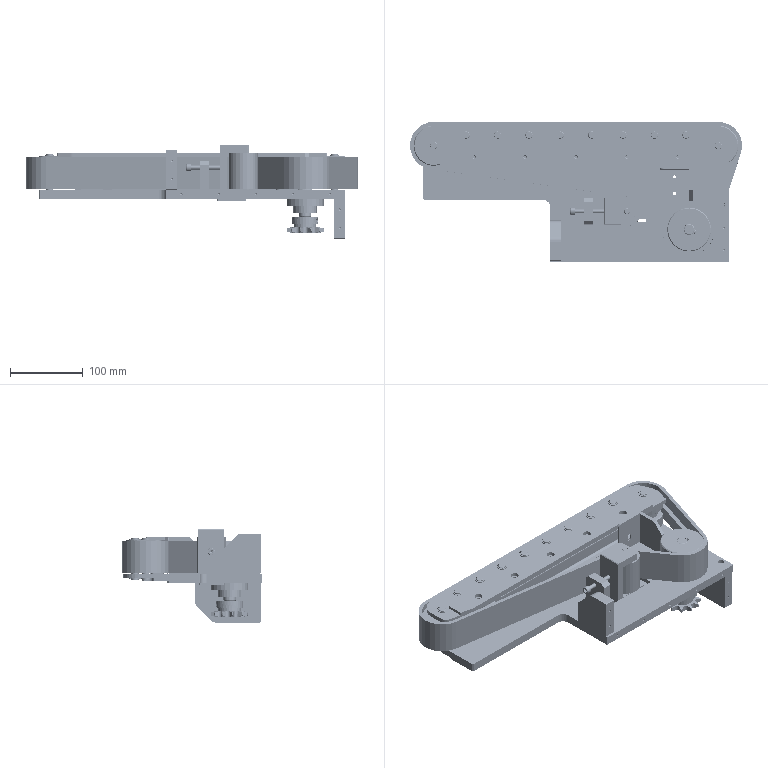Assembly | SolidWorks | mm | 100 component files | 101 solids | 6220 faces | box 455 x 192 x 128 mm | volume 1908277 mm3 | cylinder 1858 | cone 1700 | spline 1602 | plane 1058 | torus 2 | commonest cylinder face diameters 10 x162 22.2 x112 14.2 x112 14.6 x112 20.8 x112 14.8 x112 13.3 x112 13.9 x112
Bill of materials:
170423A4-AHC21-308-M5 | 11 |  | Small block. The lower body has angled (chamfered) long sides, so the end view is a trapezoid. Two diagonally opposite corners are rounded in plan. A narrower raised rib on top carries a through hole with a chamfered or countersunk entry.
170423A4-AOB02-H3045M-L320 | 1 |  | Long straight extrusion with a rectangular, roughly 1:2 cross-section. It has undercut slots on one long side and on both short sides, a closed flat opposite long side, internal cavities, and a central bore with four notches. One end is machined, with the slot features cut back and a shallow taper.
170423A4-Belt | 1 |  | Thin-walled closed band of constant height and wall thickness. In plan it is an irregular, roughly triangular or boot-shaped loop with one long straight edge, a long angled edge, an inward kink, and rounded corners.
170423A4-AdjustmentBlock2 | 1 |  | Thick rectangular plate with both top corners chamfered at 45 degrees and one round through hole centred near the top edge.
170423A4-ConveyorBeltIdlerFixture1 | 1 |  | C-shaped (channel) bracket made of a back wall and two parallel flanges. Each flange has a large through hole, the lower flange also has two small holes, and a small hole enters the edge of the upper flange. The outer corners at the flange tips are chamfered.
170423A4-ENN02-D40-L50 | 1 |  | Solid cylinder with a small coaxial through hole. A faint concentric circular edge on the end face may mark a very shallow step, recess, or face split.
170423A4-IdlerFixedAxis1 | 1 |  | Slender cylindrical pin with chamfered ends and one circumferential groove near one end, forming a short collar at the tip.
170423A4-M6X40StainlessSteelCupHeadHexSocket | 1 |  | Headed pin: a short cylindrical head with rounded edges on a long, smooth cylindrical shank with a chamfered tip.
170423A4-HI_BAY6803ZZ | 2 |  | Annular ring with a rectangular section and rounded edges. The end face shows several concentric grooves or steps between the inner and outer diameters.
170423A4-HI_BFY01-6803ZZ-L30S | 1 |  | Flanged cylindrical hub. A central sleeve passes through a thicker circular flange with four equally spaced through holes. The bore has an internal step (counterbore) at one end.
170423A4-Key5x12 | 1 |  | Prismatic bar with a stadium (rounded-end) profile and small edge chamfers. Overall it is a short block with flat parallel faces.
170423A4-Key5x30 | 1 |  | Thin prismatic bar with a stadium (rounded-end) profile and small edge chamfers. It is similar to the previous part but narrower relative to its length.
170423A4-Pulley2 | 1 |  | Spool-shaped solid of revolution: two equal chamfered flanges joined by a smaller-diameter hub that forms a wide circumferential groove, with a through-bore that has one keyway notch.
170423A4-PulleyFixedAxis1 | 1 |  | Stepped cylindrical shaft with a thin raised collar at one step, a longer plain section and a reduced-diameter end section. Both end sections have a closed-end keyway slot.
170423A4-VLF02-40-11-D15 | 1 |  | Toothed sprocket-like wheel with 12 teeth and an integral raised cylindrical hub on one side. It has a keyed central bore and radial cross holes in the hub.
170423A4-AxisCollar | 8 |  | Plain cylindrical tube or sleeve with a uniform wall and small chamfers on the ends.
170423A4-BAY6000ZZ | 28 |  | Short annular body with concentric outer and inner rings separated by a recessed ring face on each side. It looks like a shielded ball bearing envelope.
170423A4-IdlerAxis1 | 10 |  | Slender solid cylindrical pin with a narrow circumferential groove near each end and chamfered end faces.
170423A4-TBP01-10 | 20 |  | Thin flat open ring with two lugs at the split. Each lug has a small round hole, which matches the shape of an external retaining ring.
170423A4-ProfileSupportBlock | 1 |  | Bent sheet bracket with a flat base flange, a vertical back wall and a vertical side wall that has a chamfered top corner. The faces carry round holes and an oblong slot.
170423A4-Pulley1 | 2 |  | Spool-shaped solid of revolution like unnamed part: two chamfered flanges and a reduced central neck. It has a stepped (counterbored) central through-bore and no keyway.
170423A4-PulleyPlateSupportBlock1 | 1 |  | Rectangular thick plate/block with one corner cut off by a large angled chamfer that blends with fillets. It has small holes in two of its narrow edge faces.
170423A4-PulleyPlateSupportBlock2 | 1 |  | Thick plate/block similar to unnamed part but more compact. One corner has a large angled cut with large rounded blends, and two small holes are in one narrow edge face.
170423A4-PulleyRetainingPlate1 | 1 |  | Large flat plate with an L-shaped/notched outline and rounded corners. It is perforated by a row of larger holes, many small holes, one large circular cut-out and two elongated slots, and has shallow grooves or pockets on the top face.
170423A4-PulleyRetainingPlate2 | 1 |  | Long, narrow flat bar with a row of evenly spaced holes. Each end has a thinner stepped tab, and both ends carry a single hole.
170423A4-RetainingPlate1 | 1 |  | Flat rectangular plate, close to square, with uniform thickness, four chamfered corners and four round through holes in a rectangular pattern near the corners.
Mates:
1. distance | 170423A4-PulleyAssembly-1/170423A4-Pulley1-1 face at (-250.246, -5.788, 421.5) dir (0, 0, -1) | 170423A4-PulleyRetainingPlate1-1 face at (-55.246, -165.288, 421) dir (0, 0, 1)
2. concentric | 170423A4-PulleyRetainingPlate1-1 face at (-250.246, -5.788, 421) dir (0, 0, 1) r 5 | 170423A4-PulleyAssembly-1/170423A4-Pulley1-1 face at (-250.246, -5.788, 460.5) dir (0, 0, -1) r 27.5
3. coincident | 170423A4-PulleyRetainingPlate1-1 face at (-265.246, -165.288, 421) dir (-1, 0, 0) | 170423A4-PulleyRetainingPlate2-1 face at (-265.246, -36.288, 467) dir (-1, 0, 0)
4. concentric | 170423A4-PulleyAssembly-1/170423A4-Pulley1-1 face at (-250.246, -5.788, 460.5) dir (0, 0, -1) r 27.5 | 170423A4-Belt-1 face at (-250.246, -5.788, 466.5) dir (0, 0, -1) r 27.5
5. width | 170423A4-PulleyRetainingPlate1-1 face at (154.754, -165.288, 421) dir (1, 0, 0) | 170423A4-PulleyRetainingPlate1-1 face at (-265.246, -165.288, 421) dir (-1, 0, 0) | 170423A4-AOB02-H3045M-L320-1 face at (-215.246, -34.788, 420) dir (-1, 0, 0) | 170423A4-AOB02-H3045M-L320-1 face at (104.754, -34.788, 420) dir (1, 0, 0)
6. distance | 170423A4-PulleyAssembly-1/170423A4-Pulley1-1 face at (-250.246, -5.788, 460.5) dir (0, 0, 1) | 170423A4-PulleyRetainingPlate2-1 face at (-55.246, -36.288, 461) dir (0, 0, -1)
7. coincident | 170423A4-PulleyRetainingPlate1-1 face at (-215.346, -36.288, 418.5) dir (0, 1, 0) | 170423A4-AOB02-H3045M-L320-1 face at (104.754, -36.288, 420) dir (0, -1, 0)
8. coincident | 170423A4-PulleyRetainingPlate1-1 face at (-55.246, -165.288, 418.5) dir (0, 0, 1) | 170423A4-AOB02-H3045M-L320-1 face at (104.754, -7.788, 418.5) dir (0, 0, -1)
9. concentric | 170423A4-PulleyRetainingPlate1-1 face at (-205.746, 8.712, 421) dir (0, 0, 1) r 5 | 170423A4-IdlerAssembly5-1/170423A4-IdlerAxis1-1 face at (-205.746, 8.712, 470) dir (0, 0, -1) r 5
10. coincident | 170423A4-AOB02-H3045M-L320-1 face at (104.754, -25.388, 461.5) dir (0, 0, -1) | 170423A4-AHC21-308-M5-1 face at (-195.246, -17.038, 461.5) dir (0, 0, 1)
11. coincident | 170423A4-AOB02-H3045M-L320-1 face at (104.754, -29.538, 420.5) dir (0, 0, 1) | 170423A4-AHC21-308-M5-15 face at (84.754, -17.038, 420.5) dir (0, 0, -1)
12. concentric | 170423A4-AHC21-308-M5-15 face at (84.754, -21.288, 425.5) dir (0, 0, -1) r 2.067 | 170423A4-PulleyRetainingPlate1-1 face at (84.754, -21.288, 411) dir (0, 0, -1) r 5.5
13. parallel | 170423A4-AOB02-H3045M-L320-1 face at (-215.246, -34.788, 420) dir (-1, 0, 0) | 170423A4-AHC21-308-M5-15 face at (80.754, -29.538, 420.5) dir (-1, 0, 0)
14. parallel | 170423A4-AOB02-H3045M-L320-1 face at (-215.246, -34.788, 420) dir (-1, 0, 0) | 170423A4-AHC21-308-M5-1 face at (-199.246, -13.038, 461.5) dir (-1, 0, 0)
15. coincident | 170423A4-PulleyRetainingPlate1-1 face at (-55.246, -165.288, 409) dir (0, 0, -1) | 170423A4-ConveyorSynchronousPulleyAssembly-1/170423A4-BFY01-6803ZZ-L30-1/170423A4-HI_BFY01-6803ZZ-L30S-1 face at (99.754, -136.888, 409) dir (0, 0, 1)
16. concentric | 170423A4-PulleyRetainingPlate1-1 face at (99.754, -120.788, 421) dir (0, 0, -1) r 16.25 | 170423A4-ConveyorSynchronousPulleyAssembly-1/170423A4-BFY01-6803ZZ-L30-1/170423A4-HI_BFY01-6803ZZ-L30S-1 face at (99.754, -120.788, 349) dir (0, 0, 1) r 16
17. parallel | 170423A4-PulleyRetainingPlate1-1 face at (154.754, -165.288, 421) dir (1, 0, 0) | 170423A4-ConveyorSynchronousPulleyAssembly-1/170423A4-BFY01-6803ZZ-L30-1 plane at (99.754, -120.788, 399) dir (-1, 0, 0)
18. parallel | 170423A4-PulleyRetainingPlate2-1 face at (-265.246, -36.288, 467) dir (-1, 0, 0) | 170423A4-IdlerAssembly5-1/170423A4-TBP01-10-2 face at (-208.246, 15.862, 468.25) dir (-1, 0, 0)
19. parallel | 170423A4-PulleyAssembly-1/170423A4-TBP01-10-2 face at (-252.746, 1.362, 468.4) dir (-1, 0, 0) | 170423A4-PulleyRetainingPlate2-1 face at (-265.246, -36.288, 467) dir (-1, 0, 0)
20. coincident | 170423A4-PulleyRetainingPlate1-1 face at (-55.246, -165.288, 409) dir (0, 0, -1) | 170423A4-PulleyPlateSupportBlock1-1 face at (154.754, -163.288, 409) dir (0, 0, 1)
21. coincident | 170423A4-PulleyRetainingPlate1-1 face at (154.754, -165.288, 421) dir (1, 0, 0) | 170423A4-PulleyPlateSupportBlock1-1 face at (154.754, -163.288, 409) dir (1, 0, 0)
22. distance | 170423A4-PulleyPlateSupportBlock1-1 face at (154.754, -163.288, 409) dir (0, -1, 0) | 170423A4-PulleyRetainingPlate1-1 face at (-265.246, -165.288, 421) dir (0, -1, 0)
23. coincident | 170423A4-PulleyRetainingPlate2-1 face at (104.854, -6.288, 463.5) dir (0, -1, 0) | 170423A4-AOB02-H3045M-L320-1 face at (104.754, -6.288, 462) dir (0, 1, 0)
24. parallel | 170423A4-PulleyRetainingPlate1-1 face at (-265.246, 24.712, 421) dir (0, 1, 0) | 170423A4-Belt-1 face at (-250.246, 26.712, 466.5) dir (0, 1, 0)
25. coincident | 170423A4-PulleyAssembly-1/170423A4-Pulley1-1 face at (-250.246, -5.788, 421.5) dir (0, 0, -1) | 170423A4-Belt-1 face at (-250.246, -5.788, 421.5) dir (0, 0, -1)
26. distance | 170423A4-IdlerAssembly5-1/170423A4-IdlerAxis1-1 face at (-205.746, 8.712, 412) dir (0, 0, -1) | 170423A4-PulleyRetainingPlate1-1 face at (-55.246, -165.288, 415) dir (0, 0, -1)
27. concentric | 170423A4-PulleyRetainingPlate2-1 face at (-195.246, -21.288, 471) dir (0, 0, 1) r 5.5 | 170423A4-AHC21-308-M5-1 face at (-195.246, -21.288, 456.5) dir (0, 0, 1) r 2.067
28. coincident | 170423A4-PulleyRetainingPlate1-1 face at (-55.246, -165.288, 415) dir (0, 0, 1) | 170423A4-ConveyorBeltIdlerAssembly1-1/170423A4-ConveyorBeltIdlerFixture1-1 face at (-17.246, -113.788, 415) dir (0, 0, -1)
29. coincident | 170423A4-PulleyRetainingPlate1-1 face at (-44.246, -77.688, 415) dir (1, 0, 0) | 170423A4-ConveyorBeltIdlerAssembly1-1/170423A4-AdjustmentBlock2-1 face at (-44.246, -95.788, 415) dir (-1, 0, 0)
30. width | 170423A4-PulleyRetainingPlate1-1 face at (-44.246, -77.688, 415) dir (0, -1, 0) | 170423A4-PulleyRetainingPlate1-1 face at (-44.246, -113.888, 415) dir (0, 1, 0) | 170423A4-ConveyorBeltIdlerAssembly1-1/170423A4-AdjustmentBlock2-1 face at (-32.246, -77.788, 415) dir (0, 1, 0) | 170423A4-ConveyorBeltIdlerAssembly1-1/170423A4-AdjustmentBlock2-1 face at (-32.246, -113.788, 415) dir (0, -1, 0)
31. coincident | 170423A4-PulleyRetainingPlate1-1 face at (-55.246, -165.288, 421) dir (0, 0, 1) | 170423A4-ProfileSupportBlock-1 face at (59.754, -36.288, 421) dir (0, 0, -1)
32. coincident | 170423A4-AOB02-H3045M-L320-1 face at (104.754, -36.288, 447.1) dir (0, -1, 0) | 170423A4-ProfileSupportBlock-1 face at (59.754, -36.288, 421) dir (0, 1, 0)
33. coincident | 170423A4-AOB02-H3045M-L320-1 face at (104.754, -34.788, 420) dir (1, 0, 0) | 170423A4-ProfileSupportBlock-1 face at (104.754, -38.788, 423.5) dir (1, 0, 0)
34. coincident | 170423A4-PulleyRetainingPlate1-1 face at (-55.246, -165.288, 421) dir (0, 0, 1) | 170423A4-PulleyPlateSupportBlock2-1 face at (-90.246, -163.288, 421) dir (0, 0, -1)
35. coincident | 170423A4-PulleyRetainingPlate1-1 face at (-90.246, -165.288, 409) dir (-1, 0, 0) | 170423A4-PulleyPlateSupportBlock2-1 face at (-90.246, -163.288, 421) dir (-1, 0, 0)
36. coincident | 170423A4-PulleyPlateSupportBlock1-1 face at (154.754, -163.288, 409) dir (0, -1, 0) | 170423A4-PulleyPlateSupportBlock2-1 face at (-90.246, -163.288, 421) dir (0, -1, 0)
37. coincident | 170423A4-AOB02-H3045M-L320-1 face at (104.754, -30.288, 451.25) dir (0, 1, 0) | 170423A4-AHC21-308-M5-20 face at (79.754, -30.288, 445.25) dir (0, -1, 0)
38. distance | 170423A4-AHC21-308-M5-20 face at (83.754, -30.288, 432.75) dir (1, 0, 0) | 170423A4-AOB02-H3045M-L320-1 face at (104.754, -34.788, 420) dir (1, 0, 0)
39. width | 170423A4-AOB02-H3045M-L320-1 face at (104.754, -26.288, 451.25) dir (0, 0, -1) | 170423A4-AOB02-H3045M-L320-1 face at (104.754, -30.288, 430.75) dir (0, 0, 1) | 170423A4-AHC21-308-M5-20 face at (79.754, -30.288, 449.25) dir (0, 0, 1) | 170423A4-AHC21-308-M5-20 face at (79.754, -30.288, 432.75) dir (0, 0, -1)
40. coincident | 170423A4-PulleyRetainingPlate1-1 face at (-55.246, -165.288, 409) dir (0, 0, -1) | 170423A4-RetainingPlate1-1 face at (-1.246, -95.788, 409) dir (0, 0, 1)
41. concentric | 170423A4-ConveyorBeltIdlerAssembly1-1/170423A4-ConveyorBeltIdlerFixture1-1 face at (-11.246, -83.288, 415) dir (0, 0, -1) r 1.65 | 170423A4-RetainingPlate1-1 face at (-11.246, -83.288, 409) dir (0, 0, 1) r 2.25
42. concentric | 170423A4-ConveyorBeltIdlerAssembly1-1/170423A4-ConveyorBeltIdlerFixture1-1 face at (-11.246, -108.288, 415) dir (0, 0, -1) r 1.65 | 170423A4-RetainingPlate1-1 face at (-11.246, -108.288, 409) dir (0, 0, 1) r 2.25
43. concentric | 170423A4-ConveyorBeltIdlerFixture1-1 face at (18.247, 20.916, 94.14) dir (0, 0, 1) r 4 | 170423A4-IdlerFixedAxis1-1 face at (18.247, 20.916, 94.14) dir (0, 0, -1) r 4
44. coincident | 170423A4-ConveyorBeltIdlerFixture1-1 face at (-13.753, 2.916, 27.14) dir (0, 0, -1) | 170423A4-AdjustmentBlock2-1 face at (-28.753, 2.916, 27.14) dir (0, 0, -1)
45. distance | 170423A4-AdjustmentBlock2-1 face at (-28.753, 20.916, 27.14) dir (1, 0, 0) | 170423A4-ConveyorBeltIdlerFixture1-1 face at (-13.753, 2.916, 94.14) dir (-1, 0, 0)
46. coincident | 170423A4-ConveyorBeltIdlerFixture1-1 face at (-13.753, 2.916, 94.14) dir (0, -1, 0) | 170423A4-AdjustmentBlock2-1 face at (-28.753, 2.916, 27.14) dir (0, -1, 0)
47. coincident | 170423A4-ConveyorBeltIdlerFixture1-1 face at (-13.753, 2.916, 27.14) dir (0, 0, -1) | 170423A4-IdlerFixedAxis1-1 face at (18.247, 20.916, 27.14) dir (0, 0, -1)
48. concentric | 170423A4-IdlerFixedAxis1-1 face at (18.247, 20.916, 94.14) dir (0, 0, -1) r 4 | 170423A4-ENN02-D40-L50-1 face at (18.247, 20.916, 33.64) dir (0, 0, 1) r 4
49. coincident | 170423A4-ConveyorBeltIdlerFixture1-1 face at (26.247, 2.916, 33.64) dir (0, 0, 1) | 170423A4-ENN02-D40-L50-1 face at (27.991, 26.021, 33.64) dir (0, 0, -1)
50. coincident | 170423A4-ConveyorBeltIdlerFixture1-1 face at (-13.753, 2.916, 94.14) dir (-1, 0, 0) | 170423A4-M6X40StainlessSteelCupHeadHexSocket-1 face at (-13.753, 20.916, 63.64) dir (1, 0, 0)
51. concentric | 170423A4-AdjustmentBlock2-1 face at (-28.753, 20.916, 63.64) dir (1, 0, 0) r 3 | 170423A4-M6X40StainlessSteelCupHeadHexSocket-1 face at (-13.753, 20.916, 63.64) dir (-1, 0, 0) r 3
52. coincident | 170423A4-PulleyFixedAxis1-1 face at (4.319, 15.361, -55.329) dir (1, 0, 0) | 170423A4-Key5x12-1 face at (4.319, 15.361, -43.329) dir (-1, 0, 0)
53. concentric | 170423A4-PulleyFixedAxis1-1 face at (4.319, 15.361, -55.329) dir (1, 0, 0) r 2.5 | 170423A4-Key5x12-1 face at (8.819, 15.361, -55.329) dir (-1, 0, 0) r 2.5
54. concentric | 170423A4-PulleyFixedAxis1-1 face at (4.319, 15.361, -43.329) dir (1, 0, 0) r 2.5 | 170423A4-Key5x12-1 face at (8.819, 15.361, -43.329) dir (-1, 0, 0) r 2.5
55. concentric | 170423A4-PulleyFixedAxis1-1 face at (-0.1808, 15.361, -1.129) dir (0, 0, 1) r 7.5 | 170423A4-Pulley2-1 face at (-0.1808, 15.361, -1.129) dir (0, 0, 1) r 7.5
56. coincident | 170423A4-PulleyFixedAxis1-1 face at (-0.1808, 15.361, -1.129) dir (0, 0, 1) | 170423A4-Pulley2-1 face at (-0.1808, 15.361, -1.129) dir (0, 0, -1)
57. concentric | 170423A4-PulleyFixedAxis1-1 face at (-0.1808, 15.361, -60.329) dir (0, 0, 1) r 7.5 | 170423A4-VLF02-40-11-D15-1 face at (-0.1808, 15.361, -60.329) dir (0, 0, 1) r 7.5
58. coincident | 170423A4-PulleyFixedAxis1-1 face at (-0.1808, 15.361, -38.329) dir (0, 0, -1) | 170423A4-VLF02-40-11-D15-1 face at (-0.1808, 15.361, -38.329) dir (0, 0, 1)
59. coincident | 170423A4-Key5x12-1 face at (8.819, 12.861, -43.329) dir (0, -1, 0) | 170423A4-VLF02-40-11-D15-1 face at (5.819, 12.861, -38.329) dir (0, 1, 0)
60. coincident | 170423A4-PulleyFixedAxis1-1 face at (4.319, 15.361, 6.371) dir (1, 0, 0) | 170423A4-Key5x30-1 face at (4.319, 15.361, 6.371) dir (-1, 0, 0)
61. concentric | 170423A4-PulleyFixedAxis1-1 face at (4.319, 15.361, 6.371) dir (1, 0, 0) r 2.5 | 170423A4-Key5x30-1 face at (4.319, 15.361, 6.371) dir (1, 0, 0) r 2.5
62. concentric | 170423A4-PulleyFixedAxis1-1 face at (4.319, 15.361, 36.371) dir (1, 0, 0) r 2.5 | 170423A4-Key5x30-1 face at (4.319, 15.361, 36.371) dir (1, 0, 0) r 2.5
63. parallel | 170423A4-Pulley2-1 face at (-0.1808, 17.861, -1.129) dir (0, -1, 0) | 170423A4-Key5x30-1 face at (4.319, 17.861, 6.371) dir (0, 1, 0)
64. concentric | 170423A4-PulleyFixedAxis1-1 face at (-0.1808, 15.361, -38.329) dir (0, 0, 1) r 8.5 | 170423A4-BFY01-6803ZZ-L30-1/170423A4-HI_BAY6803ZZ-1 face at (-0.1808, 15.361, -8.329) dir (0, 0, 1) r 8.5
65. coincident | 170423A4-PulleyFixedAxis1-1 face at (-0.1808, 15.361, -3.629) dir (0, 0, -1) | 170423A4-BFY01-6803ZZ-L30-1/170423A4-HI_BFY01-6803ZZ-L30S-1 face at (-0.1808, 15.361, -3.629) dir (0, 0, 1)
66. concentric | 170423A4-IdlerAxis1-1 face at (12.836, 33.288, 77.757) dir (0, 0, -1) r 5 | 170423A4-AxisCollar-1 face at (12.836, 33.288, 58.257) dir (0, 0, -1) r 5.05
67. concentric | 170423A4-IdlerAxis1-1 face at (12.836, 33.288, 77.757) dir (0, 0, -1) r 5 | 170423A4-BAY6000ZZ-1 face at (12.836, 33.288, 29.557) dir (0, 0, 1) r 5
68. concentric | 170423A4-IdlerAxis1-1 face at (12.836, 33.288, 77.757) dir (0, 0, -1) r 5 | 170423A4-BAY6000ZZ-2 face at (12.836, 33.288, 58.557) dir (0, 0, 1) r 5
69. concentric | 170423A4-IdlerAxis1-1 face at (12.836, 33.288, 77.757) dir (0, 0, 1) r 4.65 | 170423A4-TBP01-10-1 face at (12.836, 33.288, 22.507) dir (0, 0, 1) r 4.65
70. coincident | 170423A4-IdlerAxis1-1 face at (12.836, 38.288, 22.507) dir (0, 0, -1) | 170423A4-TBP01-10-1 face at (15.636, 27.346, 22.507) dir (0, 0, 1)
71. concentric | 170423A4-IdlerAxis1-1 face at (12.836, 33.288, 77.757) dir (0, 0, 1) r 4.65 | 170423A4-TBP01-10-2 face at (12.836, 33.288, 76.007) dir (0, 0, 1) r 4.65
72. coincident | 170423A4-IdlerAxis1-1 face at (12.836, 38.288, 75.007) dir (0, 0, 1) | 170423A4-TBP01-10-2 face at (15.636, 27.346, 75.007) dir (0, 0, -1)
73. parallel | 170423A4-TBP01-10-1 face at (10.336, 27.346, 22.507) dir (-1, 0, 0) | 170423A4-TBP01-10-2 face at (10.336, 27.346, 76.007) dir (-1, 0, 0)
74. coincident | 170423A4-AxisCollar-1 face at (12.836, 33.288, 58.257) dir (0, 0, 1) | 170423A4-BAY6000ZZ-2 face at (11.553, 44.415, 58.257) dir (0, 0, -1)
75. distance | 170423A4-BAY6000ZZ-1 face at (12.939, 44.488, 29.257) dir (0, 0, -1) | 170423A4-IdlerAxis1-1 face at (12.836, 33.288, 19.757) dir (0, 0, -1)
76. concentric | 170423A4-IdlerAxis1-1 face at (12.836, 33.288, 77.757) dir (0, 0, -1) r 5 | 170423A4-BAY6000ZZ-3 face at (12.836, 33.288, 37.557) dir (0, 0, 1) r 5
77. coincident | 170423A4-BAY6000ZZ-1 face at (12.953, 45.988, 37.257) dir (0, 0, 1) | 170423A4-BAY6000ZZ-3 face at (12.939, 44.488, 37.257) dir (0, 0, -1)
78. coincident | 170423A4-AxisCollar-1 face at (12.836, 33.288, 45.257) dir (0, 0, -1) | 170423A4-BAY6000ZZ-3 face at (12.953, 45.988, 45.257) dir (0, 0, 1)
79. coincident | 170423A4-Pulley1-1 face at (0.5661, 22.017, 62.198) dir (0, 0, 1) | 170423A4-BAY6000ZZ-1 face at (0.5661, 34.717, 62.198) dir (0, 0, -1)
80. concentric | 170423A4-Pulley1-1 face at (0.5661, 22.017, 62.198) dir (0, 0, 1) r 13 | 170423A4-BAY6000ZZ-1 face at (0.5661, 22.017, 69.898) dir (0, 0, -1) r 13
81. coincident | 170423A4-Pulley1-1 face at (0.5661, 22.017, 39.198) dir (0, 0, -1) | 170423A4-BAY6000ZZ-2 face at (0.5661, 33.217, 39.198) dir (0, 0, 1)
82. concentric | 170423A4-Pulley1-1 face at (0.5661, 22.017, 31.198) dir (0, 0, 1) r 7.5 | 170423A4-BAY6000ZZ-2 face at (0.5661, 22.017, 38.898) dir (0, 0, -1) r 13
83. concentric | 170423A4-BAY6000ZZ-2 face at (0.5661, 22.017, 38.898) dir (0, 0, -1) r 5 | 170423A4-IdlerAxis1-1 face at (0.5661, 22.017, 79.698) dir (0, 0, -1) r 5
84. width | 170423A4-IdlerAxis1-1 face at (0.5661, 22.017, 21.698) dir (0, 0, -1) | 170423A4-IdlerAxis1-1 face at (0.5661, 22.017, 79.698) dir (0, 0, 1) | 170423A4-Pulley1-1 face at (0.5661, 22.017, 70.198) dir (0, 0, 1) | 170423A4-Pulley1-1 face at (0.5661, 22.017, 31.198) dir (0, 0, -1)
85. concentric | 170423A4-IdlerAxis1-1 face at (0.5661, 22.017, 79.698) dir (0, 0, 1) r 4.65 | 170423A4-TBP01-10-1 face at (0.5661, 22.017, 24.448) dir (0, 0, 1) r 4.65
86. coincident | 170423A4-IdlerAxis1-1 face at (0.5661, 27.017, 24.448) dir (0, 0, -1) | 170423A4-TBP01-10-1 face at (3.366, 16.075, 24.448) dir (0, 0, 1)
87. concentric | 170423A4-IdlerAxis1-1 face at (0.5661, 22.017, 79.698) dir (0, 0, 1) r 4.65 | 170423A4-TBP01-10-2 face at (0.5661, 22.017, 78.098) dir (0, 0, 1) r 4.65
88. coincident | 170423A4-IdlerAxis1-1 face at (0.5661, 27.017, 78.098) dir (0, 0, -1) | 170423A4-TBP01-10-2 face at (3.366, 16.075, 78.098) dir (0, 0, 1)
89. parallel | 170423A4-TBP01-10-1 face at (-1.934, 16.075, 24.448) dir (-1, 0, 0) | 170423A4-TBP01-10-2 face at (-1.934, 16.075, 78.098) dir (-1, 0, 0)